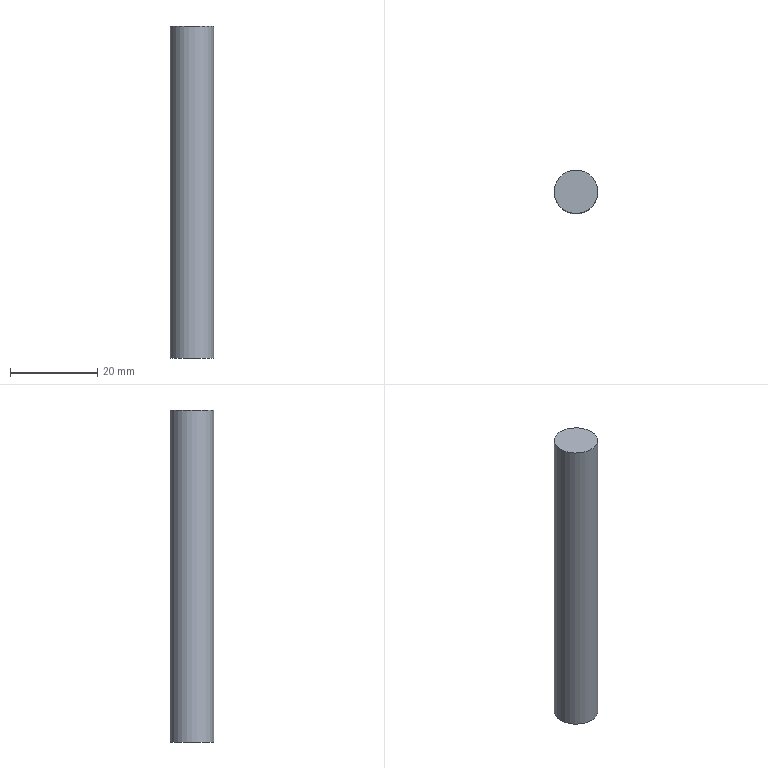Component | NX | 08__STUD_M10X1__2_2 | 1 solid | 3 faces | box 10 x 10 x 76 mm | volume 5969 mm3 | plane 2 | cylinder 1 | commonest cylinder face diameters 10 x1
STEP:
#1=CARTESIAN_POINT('',(0.,0.,0.));
#2=DIRECTION('',(0.,0.,1.));
#3=DIRECTION('',(1.,0.,0.));
#4=AXIS2_PLACEMENT_3D('',#1,#2,#3);
#5=CARTESIAN_POINT('',(36.625,-1.269,813.));
#6=VERTEX_POINT('',#5);
#7=CARTESIAN_POINT('',(31.625,-1.269,813.));
#8=DIRECTION('',(0.,0.,1.));
#9=DIRECTION('',(1.,0.,0.));
#10=AXIS2_PLACEMENT_3D('',#7,#8,#9);
#11=CIRCLE('',#10,5.);
#12=CARTESIAN_POINT('',(31.625,-1.269,813.));
#13=DIRECTION('',(0.,0.,1.));
#14=DIRECTION('',(1.,0.,0.));
#15=AXIS2_PLACEMENT_3D('',#12,#13,#14);
#16=PLANE('',#15);
#17=CARTESIAN_POINT('',(0.,0.));
#18=DIRECTION('',(1.,0.));
#19=AXIS2_PLACEMENT_2D('',#17,#18);
#20=CIRCLE('',#19,5.);
#21=(GEOMETRIC_REPRESENTATION_CONTEXT(2)PARAMETRIC_REPRESENTATION_CONTEXT()REPRESENTATION_CONTEXT('',''));
#22=DEFINITIONAL_REPRESENTATION('',(#20),#21);
#23=PCURVE('',#16,#22);
#24=CARTESIAN_POINT('',(31.625,-1.269,889.));
#25=DIRECTION('',(0.,0.,1.));
#26=DIRECTION('',(1.,0.,0.));
#27=AXIS2_PLACEMENT_3D('',#24,#25,#26);
#28=CYLINDRICAL_SURFACE('',#27,5.);
#29=CARTESIAN_POINT('',(0.,-76.));
#30=DIRECTION('',(1.,0.));
#31=VECTOR('',#30,1.);
#32=LINE('',#29,#31);
#33=(GEOMETRIC_REPRESENTATION_CONTEXT(2)PARAMETRIC_REPRESENTATION_CONTEXT()REPRESENTATION_CONTEXT('',''));
#34=DEFINITIONAL_REPRESENTATION('',(#32),#33);
#35=PCURVE('',#28,#34);
#36=SURFACE_CURVE('',#11,(#23,#35),.PCURVE_S1.);
#37=EDGE_CURVE('',#6,#6,#36,.T.);
#38=ORIENTED_EDGE('',*,*,#37,.F.);
#39=EDGE_LOOP('',(#38));
#40=FACE_BOUND('',#39,.T.);
#41=ADVANCED_FACE('',(#40),#16,.F.);
#42=CARTESIAN_POINT('',(36.625,-1.269,889.));
#43=VERTEX_POINT('',#42);
#44=CARTESIAN_POINT('',(31.625,-1.269,889.));
#45=DIRECTION('',(0.,0.,1.));
#46=DIRECTION('',(1.,0.,0.));
#47=AXIS2_PLACEMENT_3D('',#44,#45,#46);
#48=CIRCLE('',#47,5.);
#49=CARTESIAN_POINT('',(0.,0.));
#50=DIRECTION('',(1.,0.));
#51=VECTOR('',#50,1.);
#52=LINE('',#49,#51);
#53=(GEOMETRIC_REPRESENTATION_CONTEXT(2)PARAMETRIC_REPRESENTATION_CONTEXT()REPRESENTATION_CONTEXT('',''));
#54=DEFINITIONAL_REPRESENTATION('',(#52),#53);
#55=PCURVE('',#28,#54);
#56=CARTESIAN_POINT('',(31.625,3.731,889.));
#57=DIRECTION('',(0.,0.,-1.));
#58=DIRECTION('',(-1.,-0.,0.));
#59=AXIS2_PLACEMENT_3D('',#56,#57,#58);
#60=PLANE('',#59);
#61=CARTESIAN_POINT('',(-5.,-5.));
#62=CARTESIAN_POINT('',(-5.,3.66));
#63=CARTESIAN_POINT('',(2.5,-0.6699));
#64=CARTESIAN_POINT('',(10.,-5.));
#65=CARTESIAN_POINT('',(2.5,-9.33));
#66=CARTESIAN_POINT('',(-5.,-13.66));
#67=CARTESIAN_POINT('',(-5.,-5.));
#68=(BOUNDED_CURVE()B_SPLINE_CURVE(2,(#61,#62,#63,#64,#65,#66,#67),.UNSPECIFIED.,.T.,.F.)B_SPLINE_CURVE_WITH_KNOTS((1,2,2,2,2,1),(-2.094,0.,2.094,4.189,6.283,8.378),.UNSPECIFIED.)CURVE()GEOMETRIC_REPRESENTATION_ITEM()RATIONAL_B_SPLINE_CURVE((1.,0.5,1.,0.5,1.,0.5,1.))REPRESENTATION_ITEM(''));
#69=(GEOMETRIC_REPRESENTATION_CONTEXT(2)PARAMETRIC_REPRESENTATION_CONTEXT()REPRESENTATION_CONTEXT('',''));
#70=DEFINITIONAL_REPRESENTATION('',(#68),#69);
#71=PCURVE('',#60,#70);
#72=SURFACE_CURVE('',#48,(#55,#71),.PCURVE_S1.);
#73=EDGE_CURVE('',#43,#43,#72,.T.);
#74=ORIENTED_EDGE('',*,*,#73,.F.);
#75=CARTESIAN_POINT('',(36.625,-1.269,813.));
#76=CARTESIAN_POINT('',(36.625,-1.269,889.));
#77=B_SPLINE_CURVE_WITH_KNOTS('',1,(#75,#76),.UNSPECIFIED.,.F.,.F.,(2,2),(-76.,0.),.PIECEWISE_BEZIER_KNOTS.);
#78=CARTESIAN_POINT('',(0.,0.));
#79=DIRECTION('',(0.,1.));
#80=VECTOR('',#79,1.);
#81=LINE('',#78,#80);
#82=(GEOMETRIC_REPRESENTATION_CONTEXT(2)PARAMETRIC_REPRESENTATION_CONTEXT()REPRESENTATION_CONTEXT('',''));
#83=DEFINITIONAL_REPRESENTATION('',(#81),#82);
#84=PCURVE('',#28,#83);
#85=CARTESIAN_POINT('',(6.283,0.));
#86=DIRECTION('',(0.,1.));
#87=VECTOR('',#86,1.);
#88=LINE('',#85,#87);
#89=(GEOMETRIC_REPRESENTATION_CONTEXT(2)PARAMETRIC_REPRESENTATION_CONTEXT()REPRESENTATION_CONTEXT('',''));
#90=DEFINITIONAL_REPRESENTATION('',(#88),#89);
#91=PCURVE('',#28,#90);
#92=SEAM_CURVE('',#77,(#84,#91),.PCURVE_S1.);
#93=EDGE_CURVE('',#6,#43,#92,.T.);
#94=ORIENTED_EDGE('',*,*,#93,.F.);
#95=ORIENTED_EDGE('',*,*,#37,.T.);
#96=ORIENTED_EDGE('',*,*,#93,.T.);
#97=EDGE_LOOP('',(#74,#94,#95,#96));
#98=FACE_BOUND('',#97,.T.);
#99=ADVANCED_FACE('',(#98),#28,.T.);
#100=ORIENTED_EDGE('',*,*,#73,.T.);
#101=EDGE_LOOP('',(#100));
#102=FACE_BOUND('',#101,.T.);
#103=ADVANCED_FACE('',(#102),#60,.F.);
#104=CLOSED_SHELL('',(#41,#99,#103));
#105=MANIFOLD_SOLID_BREP('',#104);
#106=(LENGTH_UNIT()NAMED_UNIT(*)SI_UNIT(.MILLI.,.METRE.));
#107=UNCERTAINTY_MEASURE_WITH_UNIT(LENGTH_MEASURE(0.00001),#106,'','');
#108=(NAMED_UNIT(*)PLANE_ANGLE_UNIT()SI_UNIT($,.RADIAN.));
#109=(NAMED_UNIT(*)SI_UNIT($,.STERADIAN.)SOLID_ANGLE_UNIT());
#110=(GEOMETRIC_REPRESENTATION_CONTEXT(3)GLOBAL_UNCERTAINTY_ASSIGNED_CONTEXT((#107))GLOBAL_UNIT_ASSIGNED_CONTEXT((#106,#108,#109))REPRESENTATION_CONTEXT('',''));
#111=ADVANCED_BREP_SHAPE_REPRESENTATION('',(#4,#105),#110);